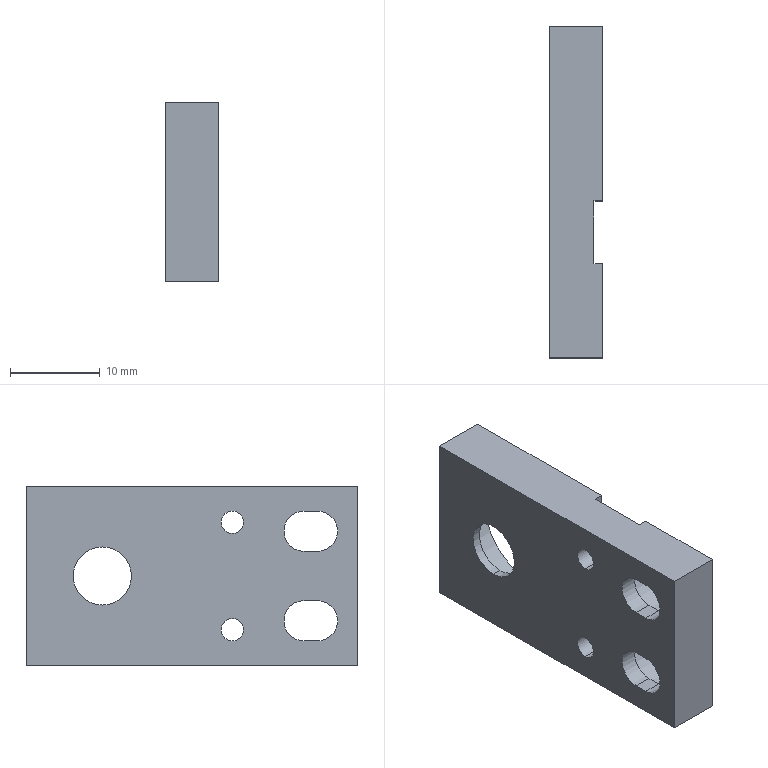Component | SolidWorks | AS-011-JG0131-1 | 1 solid | 37 faces | volume 2800 mm3 | plane 21 | cylinder 16 | commonest cylinder face diameters 2.5 x4 4.5 x4 7.5 x4 15 x2 6.5 x2